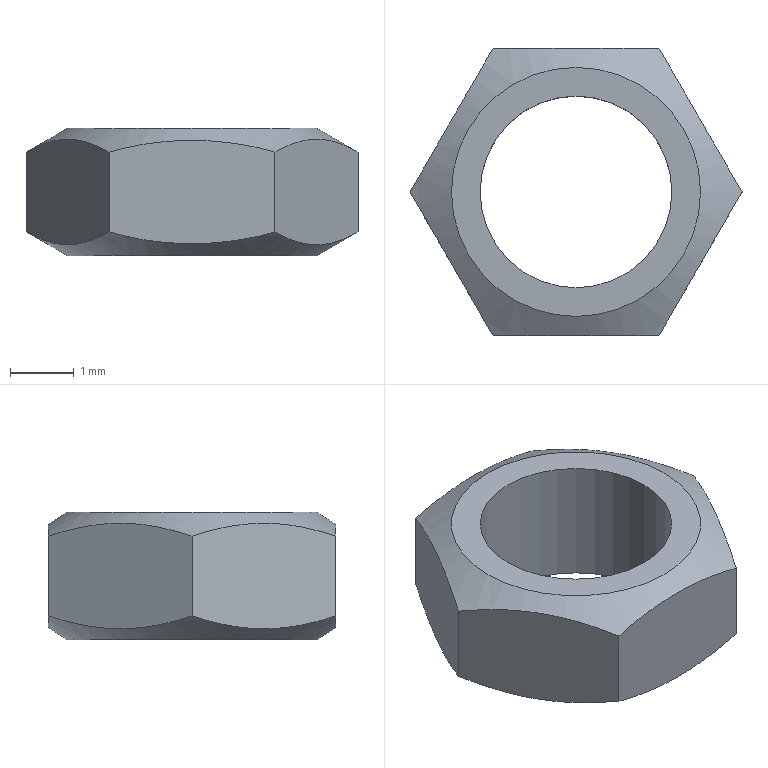Component | NX | NUT_M3 | 1 solid | 11 faces | volume 19 mm3 | plane 8 | cone 2 | cylinder 1 | commonest cylinder face diameters 3 x1